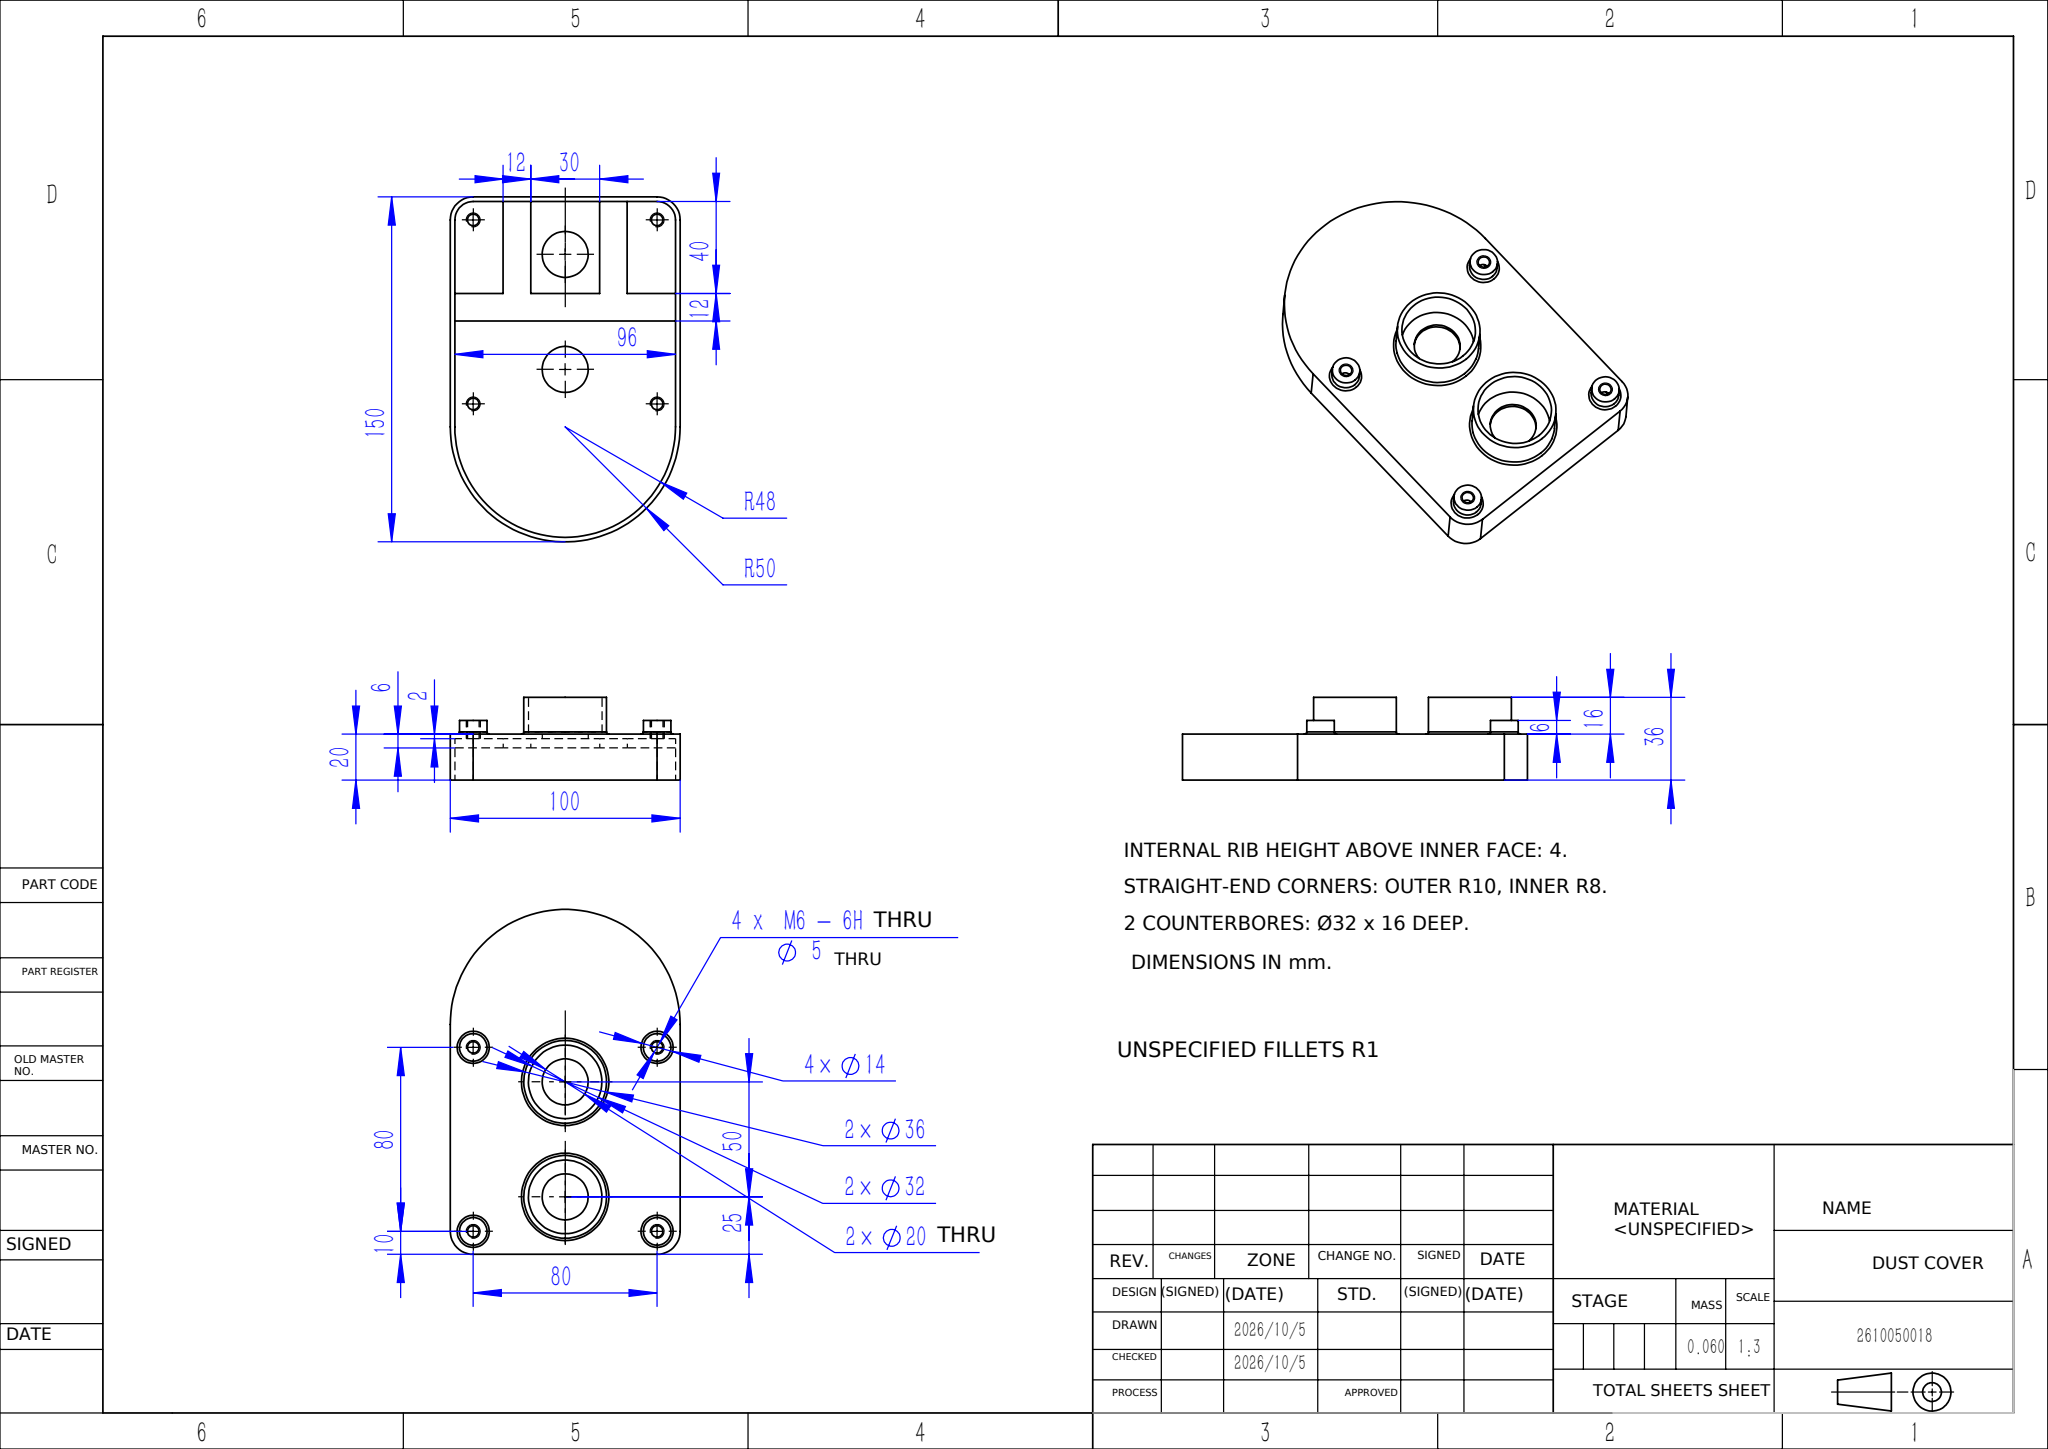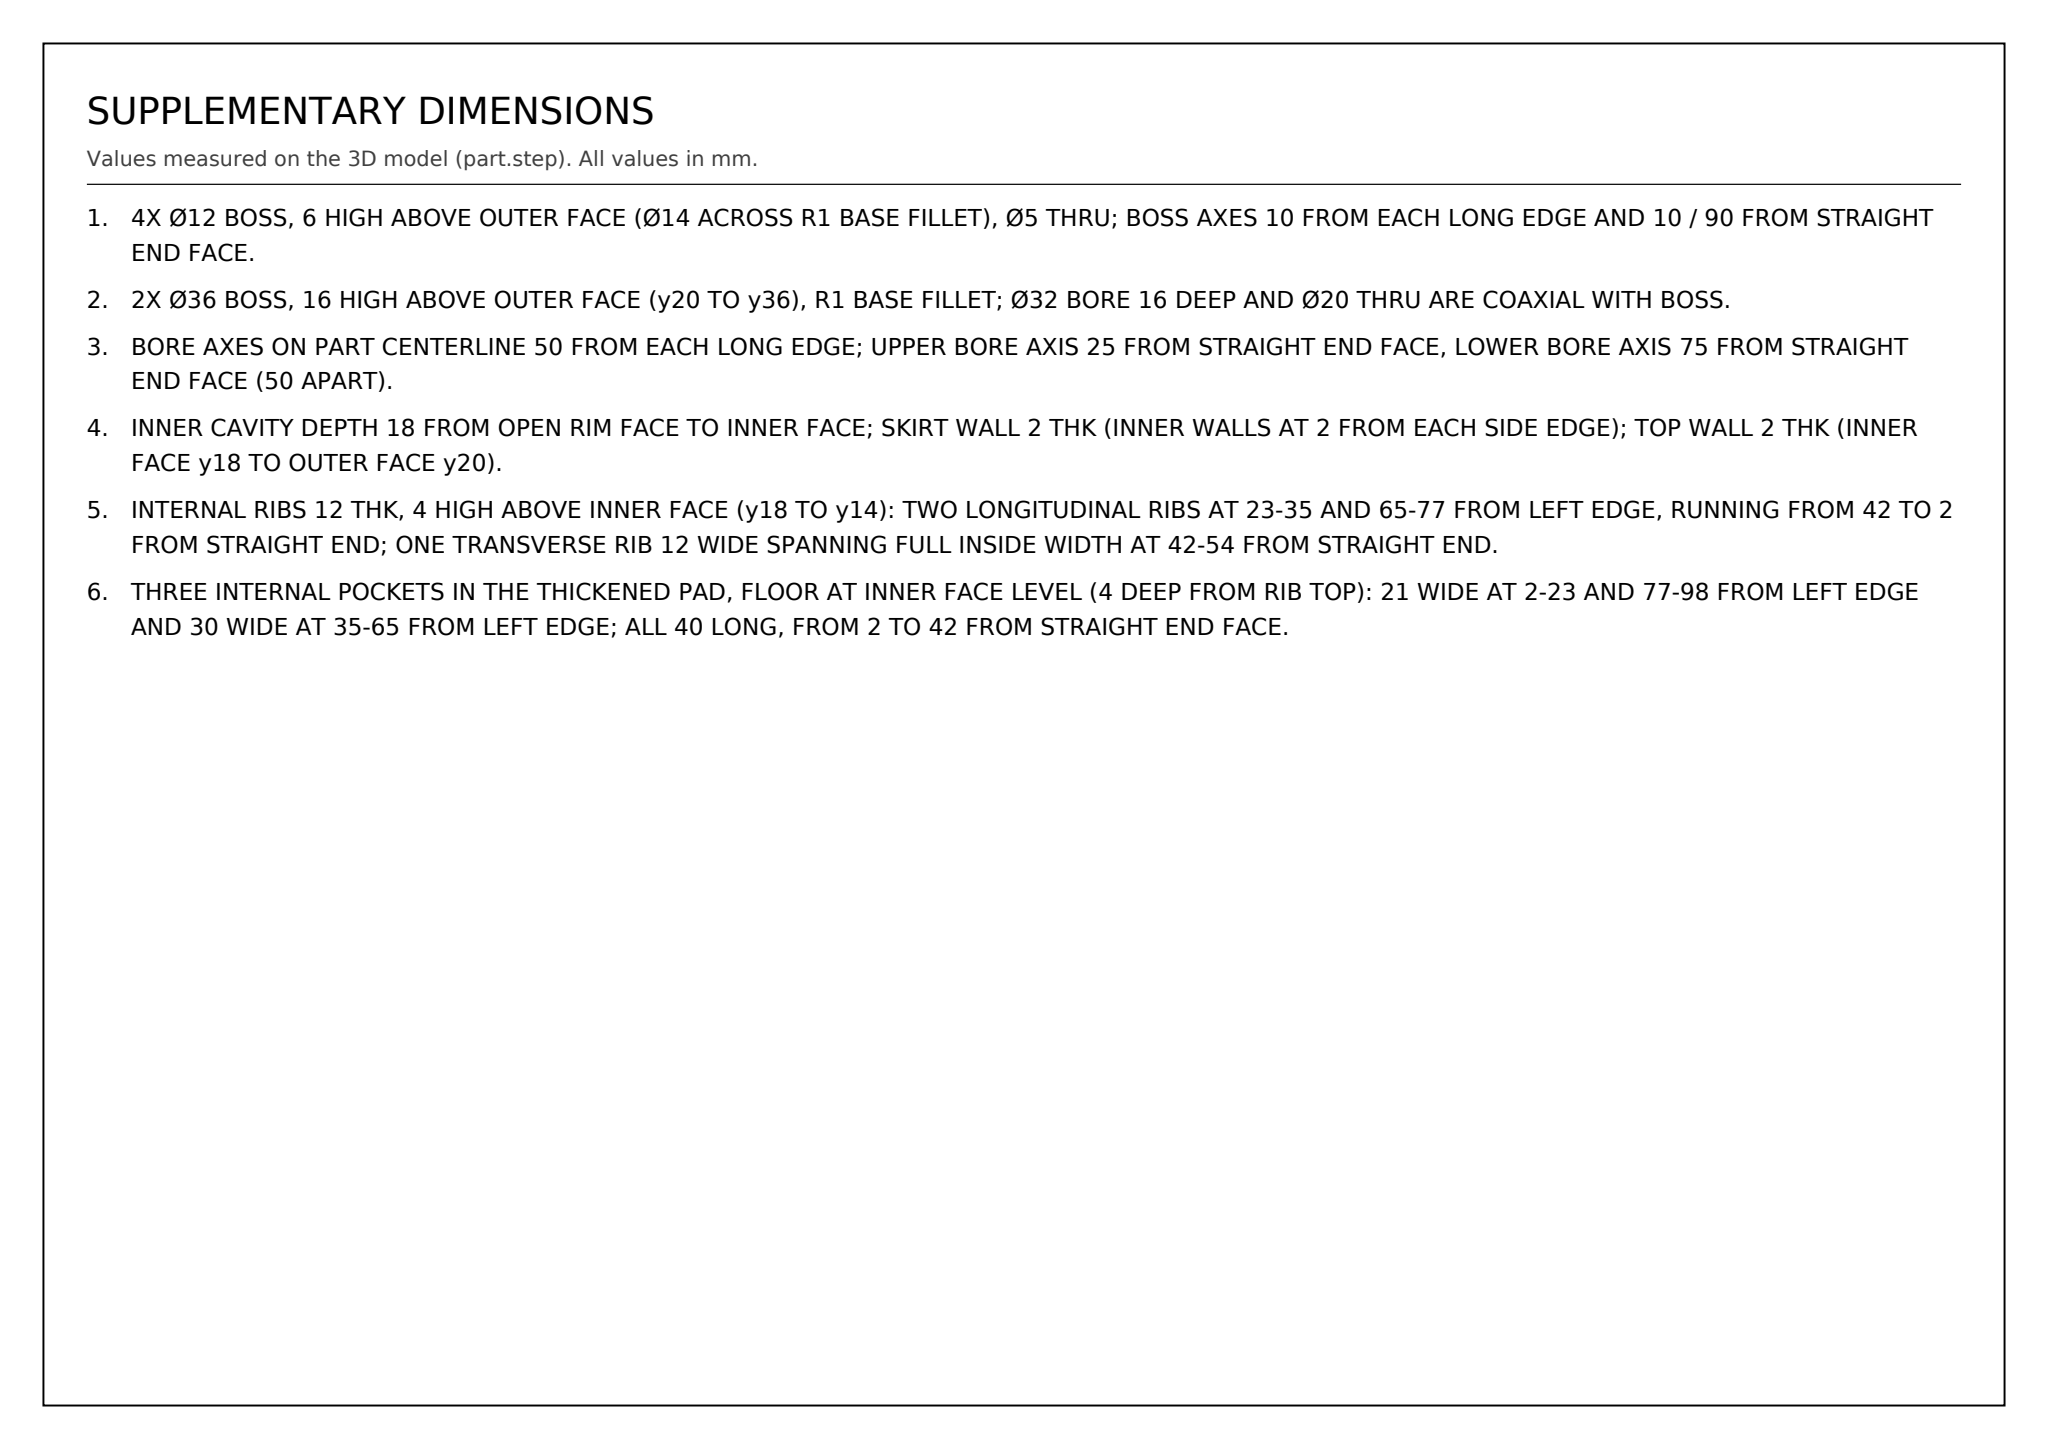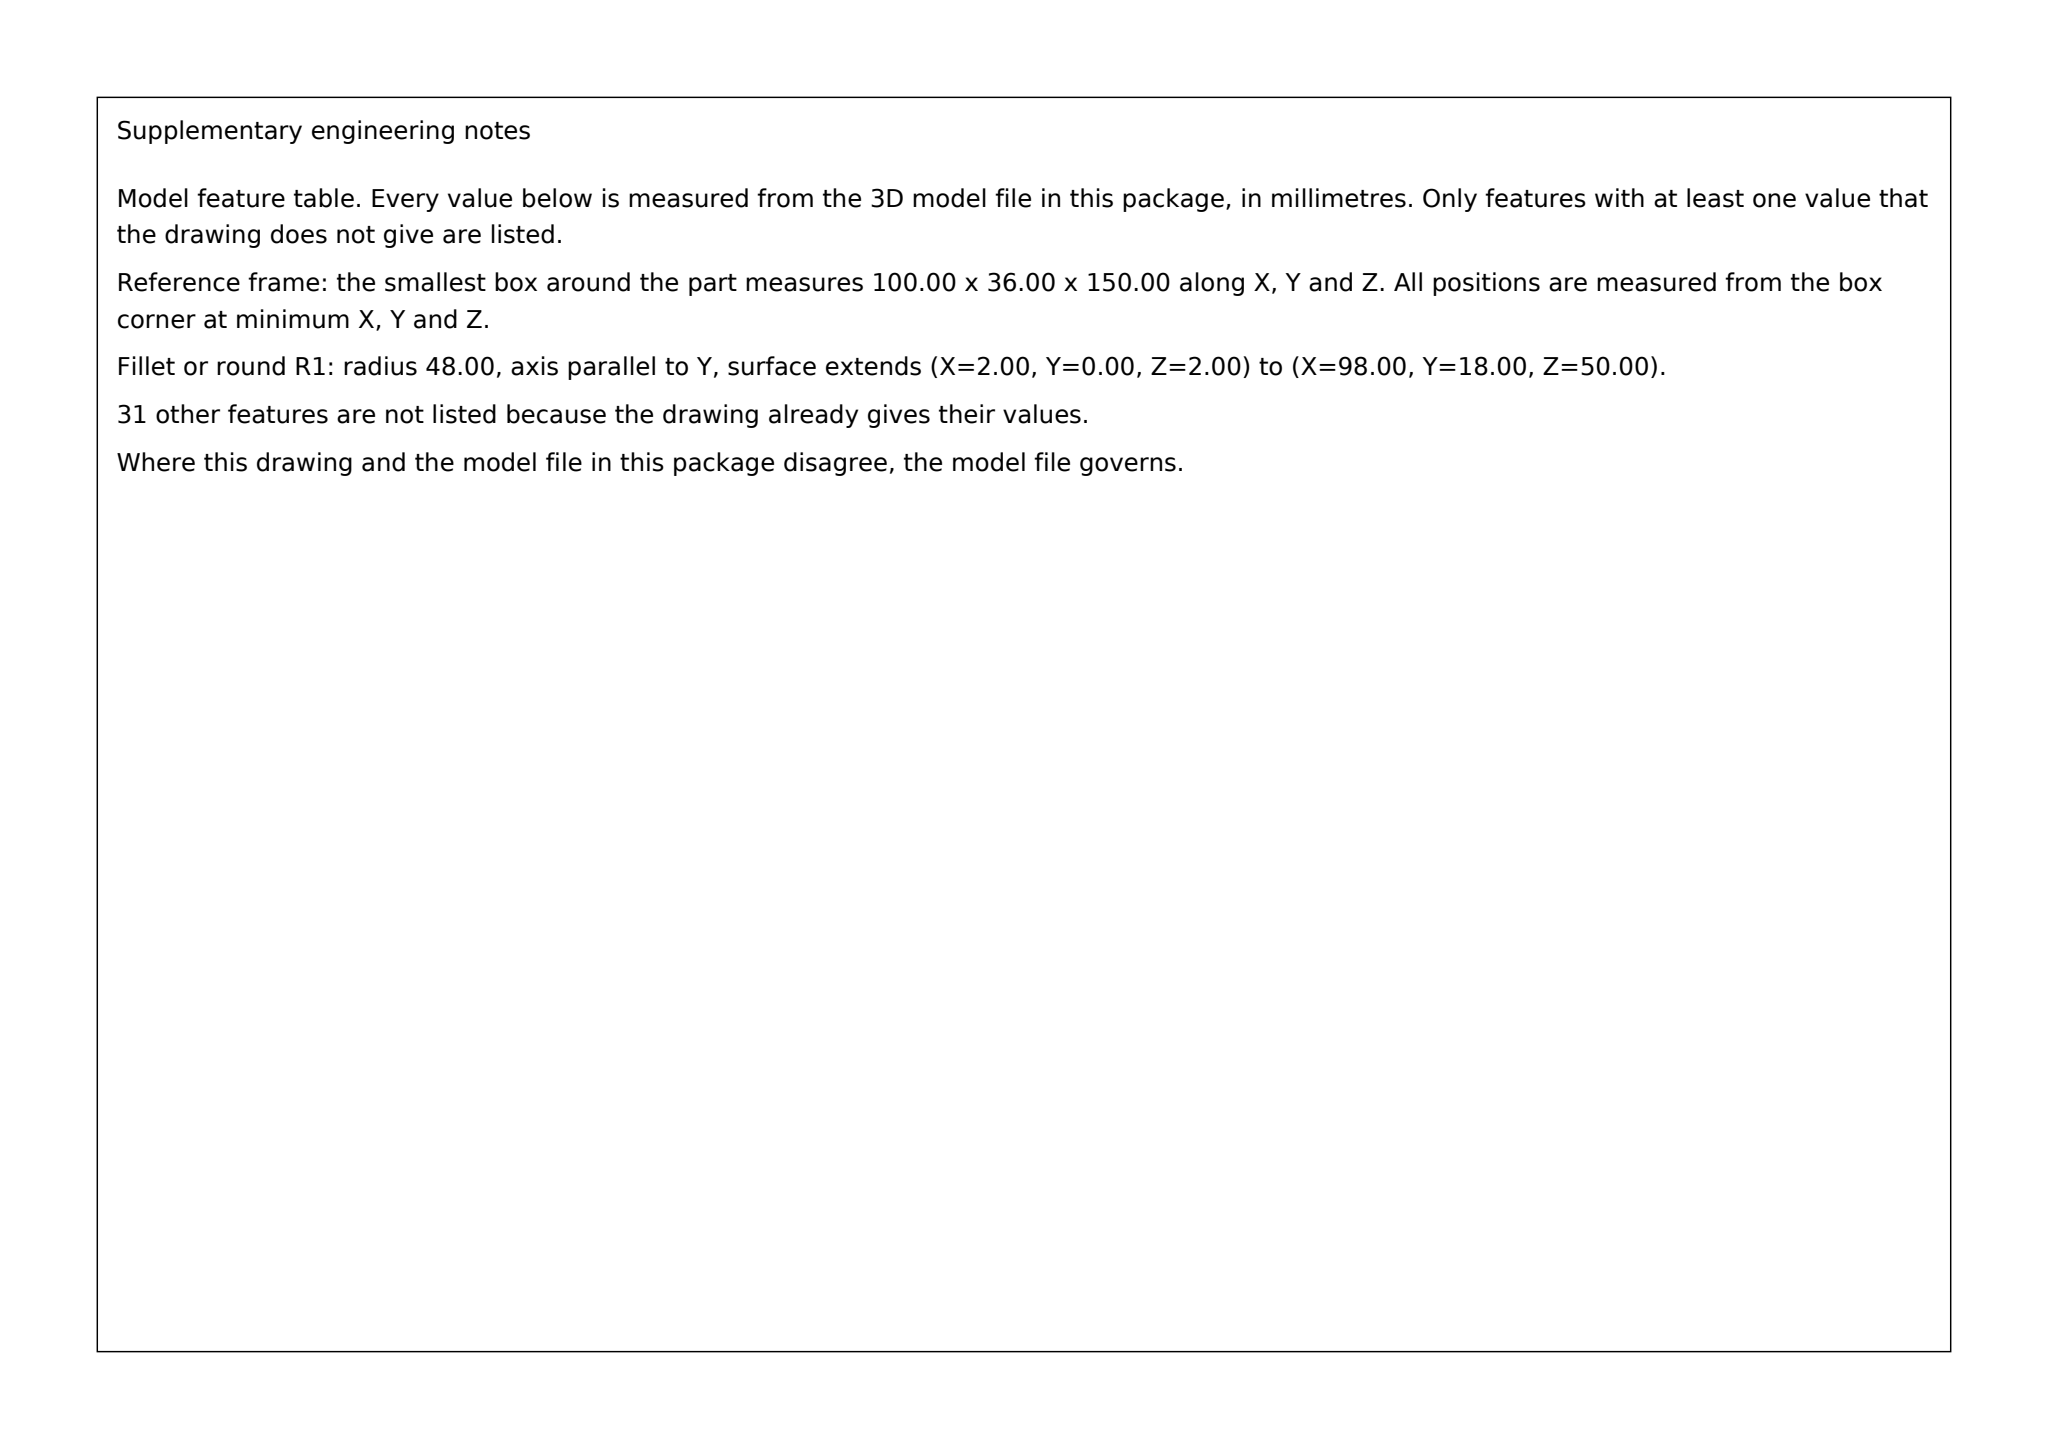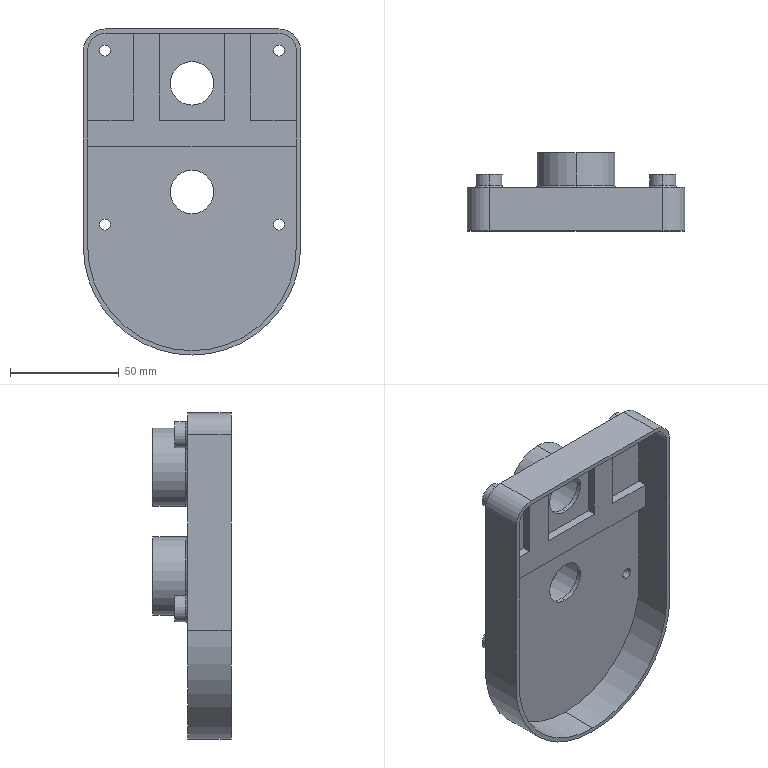Part | SolidWorks | mm | 1 solid | 77 faces | box 100 x 36 x 150 mm | volume 59884 mm3 | cylinder 36 | plane 29 | torus 12 | commonest cylinder face diameters 5 x8 12 x8 20 x6 32 x4 36 x4 96 x2 100 x2 16 x2
Drawing notes:
4X Ø12 BOSS, 6 HIGH ABOVE OUTER FACE (Ø14 ACROSS R1 BASE FILLET), Ø5 THRU; BOSS AXES 10 FROM EACH LONG EDGE AND 10 / 90 FROM STRAIGHT END FACE. | from the solid: cylinders boss/shaft Ø12 axis y from 21 to 36? (y 21->26) at (10,140),(90,140),(10,60),(90,60); hole/bore Ø5 y 18->26; tori minor_r 1.0 major 7.0 (x8)
2X Ø36 BOSS, 16 HIGH ABOVE OUTER FACE (y20 TO y36), R1 BASE FILLET; Ø32 BORE 16 DEEP AND Ø20 THRU ARE COAXIAL WITH BOSS. | from the solid: cylinders boss/shaft Ø36 axis y from 21 to 36; hole/bore Ø32 y 20->36; hole/bore Ø20 y 18->20; tori minor_r 1.0 major 19.0
BORE AXES ON PART CENTERLINE 50 FROM EACH LONG EDGE; UPPER BORE AXIS 25 FROM STRAIGHT END FACE, LOWER BORE AXIS 75 FROM STRAIGHT END FACE (50 APART). | from the solid: cylinders Ø20/Ø32/Ø36 axis y at axis_pos (50,125) and (50,75); bbox_xyz 100 x 36 x 150
INNER CAVITY DEPTH 18 FROM OPEN RIM FACE TO INNER FACE; SKIRT WALL 2 THK (INNER WALLS AT 2 FROM EACH SIDE EDGE); TOP WALL 2 THK (INNER FACE y18 TO OUTER FACE y20). | from the solid: axis_planes x 2.0 and x 98.0 extent y[0,18]; y 18.0 extent x[2,98] z[2,96] area 7682; y 0.0 rim plane; y 20.0 outer face
INTERNAL RIBS 12 THK, 4 HIGH ABOVE INNER FACE (y18 TO y14): TWO LONGITUDINAL RIBS AT 23-35 AND 65-77 FROM LEFT EDGE, RUNNING FROM 42 TO 2 FROM STRAIGHT END; ONE TRANSVERSE RIB 12 WIDE SPANNING FULL INSIDE WIDTH AT 42-54 FROM STRAIGHT END. | from the solid: axis_planes x 23/35/65/77 extent y[14,18] z[108,148] area 160; y 14.0 extent x[2,98] z[96,148] area 2112; z 108.0 planes y[14,18]
THREE INTERNAL POCKETS IN THE THICKENED PAD, FLOOR AT INNER FACE LEVEL (4 DEEP FROM RIB TOP): 21 WIDE AT 2-23 AND 77-98 FROM LEFT EDGE AND 30 WIDE AT 35-65 FROM LEFT EDGE; ALL 40 LONG, FROM 2 TO 42 FROM STRAIGHT END FACE. | from the solid: axis_planes y 18.0 extent x[2,23] z[108,148] area 807; y 18.0 extent x[35,65] z[108,148] area 886; y 18.0 extent x[77,98] z[108,148] area 807
build123d program:
from build123d import *

# Parameters (mm, degrees)
BOSS_EXTRUDE1_DEPTH = 20
FILLET1_R           = 10
SHELL1_T            = -2
SKETCH2_R           = 6
BOSS_EXTRUDE2_DEPTH = 6
M6_TAPPED_HOLE1_D   = 5
SKETCH6_R           = 18
SKETCH6_R_2         = 16
BOSS_EXTRUDE3_DEPTH = 16
SKETCH7_R           = 10
CUT_EXTRUDE1_DEPTH  = 160.374
BOSS_EXTRUDE4_DEPTH = 4
FILLET3_R           = 1


with BuildPart() as part:
    # Sketch1 → Boss-Extrude1 (new body)
    with BuildSketch(Plane(origin=(0, 0, 0), x_dir=(1, 0, 0), z_dir=(0, 1, 0))):
        with BuildLine():
            Line((-50, 100), (-50, 0))
            Line((-50, 0), (50, 0))
            Line((50, 0), (50, 100))
            ThreePointArc((50, 100), (0, 150), (-50, 100))
        make_face()
    extrude(amount=BOSS_EXTRUDE1_DEPTH)

    # Fillet1
    fillet1_edges = [part.edges().sort_by_distance(p)[0] for p in [
        (50, 10, 0),
        (-50, 10, 0),
    ]]
    fillet(fillet1_edges, radius=FILLET1_R)

    # Shell1
    shell1_openings = [part.faces().sort_by_distance(p)[0] for p in [
        (0, 0, -70.292),
    ]]
    offset(amount=SHELL1_T, openings=shell1_openings, kind=Kind.INTERSECTION)

    # Sketch2 → Boss-Extrude2 (add)
    with BuildSketch(Plane(origin=(0, 20, 0), x_dir=(1, 0, 0), z_dir=(0, 1, 0))):
        with Locations(Location((-40, 10, 0), (0, 0, 270))):
            Circle(SKETCH2_R)
        with Locations(Location((40, 10, 0), (0, 0, 270))):
            Circle(SKETCH2_R)
        with Locations(Location((40, 90, 0), (0, 0, 270))):
            Circle(SKETCH2_R)
        with Locations(Location((-40, 90, 0), (0, 0, 270))):
            Circle(SKETCH2_R)
    extrude(amount=BOSS_EXTRUDE2_DEPTH)

    # M6 Tapped Hole1 (through all)
    with Locations(Plane(origin=(0, 26, 0), x_dir=(1, 0, 0), z_dir=(0, 1, 0))):
        with Locations((-40, 90), (40, 90), (-40, 10), (40, 10)):
            Hole(M6_TAPPED_HOLE1_D / 2)

    # Sketch6 → Boss-Extrude3 (add)
    # profile 1 of 2: a face of its own
    with BuildSketch(Plane(origin=(0, 20, 0), x_dir=(1, 0, 0), z_dir=(0, 1, 0))):
        with Locations(Location((0, 25, 0), (0, 0, 270))):
            Circle(SKETCH6_R)
        with Locations(Location((0, 25, 0), (0, 0, 270))):
            Circle(SKETCH6_R_2, mode=Mode.SUBTRACT)
    # profile 2 of 2: a face of its own
    with BuildSketch(Plane(origin=(0, 20, 0), x_dir=(1, 0, 0), z_dir=(0, 1, 0))):
        with Locations(Location((0, 75, 0), (0, 0, 270))):
            Circle(SKETCH6_R)
        with Locations(Location((0, 75, 0), (0, 0, 270))):
            Circle(SKETCH6_R_2, mode=Mode.SUBTRACT)
    extrude(amount=BOSS_EXTRUDE3_DEPTH)

    # Sketch7 → Cut-Extrude1 (cut, through all)
    with BuildSketch(Plane(origin=(0, 20, 0), x_dir=(1, 0, 0), z_dir=(0, 1, 0))):
        with Locations(Location((0, 75, 0), (0, 0, 270))):
            Circle(SKETCH7_R)
        with Locations(Location((0, 25, 0), (0, 0, 270))):
            Circle(SKETCH7_R)
    extrude(amount=-CUT_EXTRUDE1_DEPTH, mode=Mode.SUBTRACT)

    # Sketch8 → Boss-Extrude4 (add)
    with BuildSketch(Plane.XZ.offset(-18)):
        Polygon((-48, -42), (-27, -42), (-27, -2), (-15, -2), (-15, -42), (15, -42), (15, -2), (27, -2), (27, -42), (48, -42), (48, -54), (-48, -54), align=None)
    extrude(amount=BOSS_EXTRUDE4_DEPTH)

    # Fillet3
    fillet3_edges = [part.edges().sort_by_distance(p)[0] for p in [
        (-40, 20, -96),
        (40, 20, -96),
        (40, 20, -16),
        (-40, 20, -16),
        (0, 20, -43),
        (0, 20, -93),
    ]]
    fillet(fillet3_edges, radius=FILLET3_R)


solid = part.part